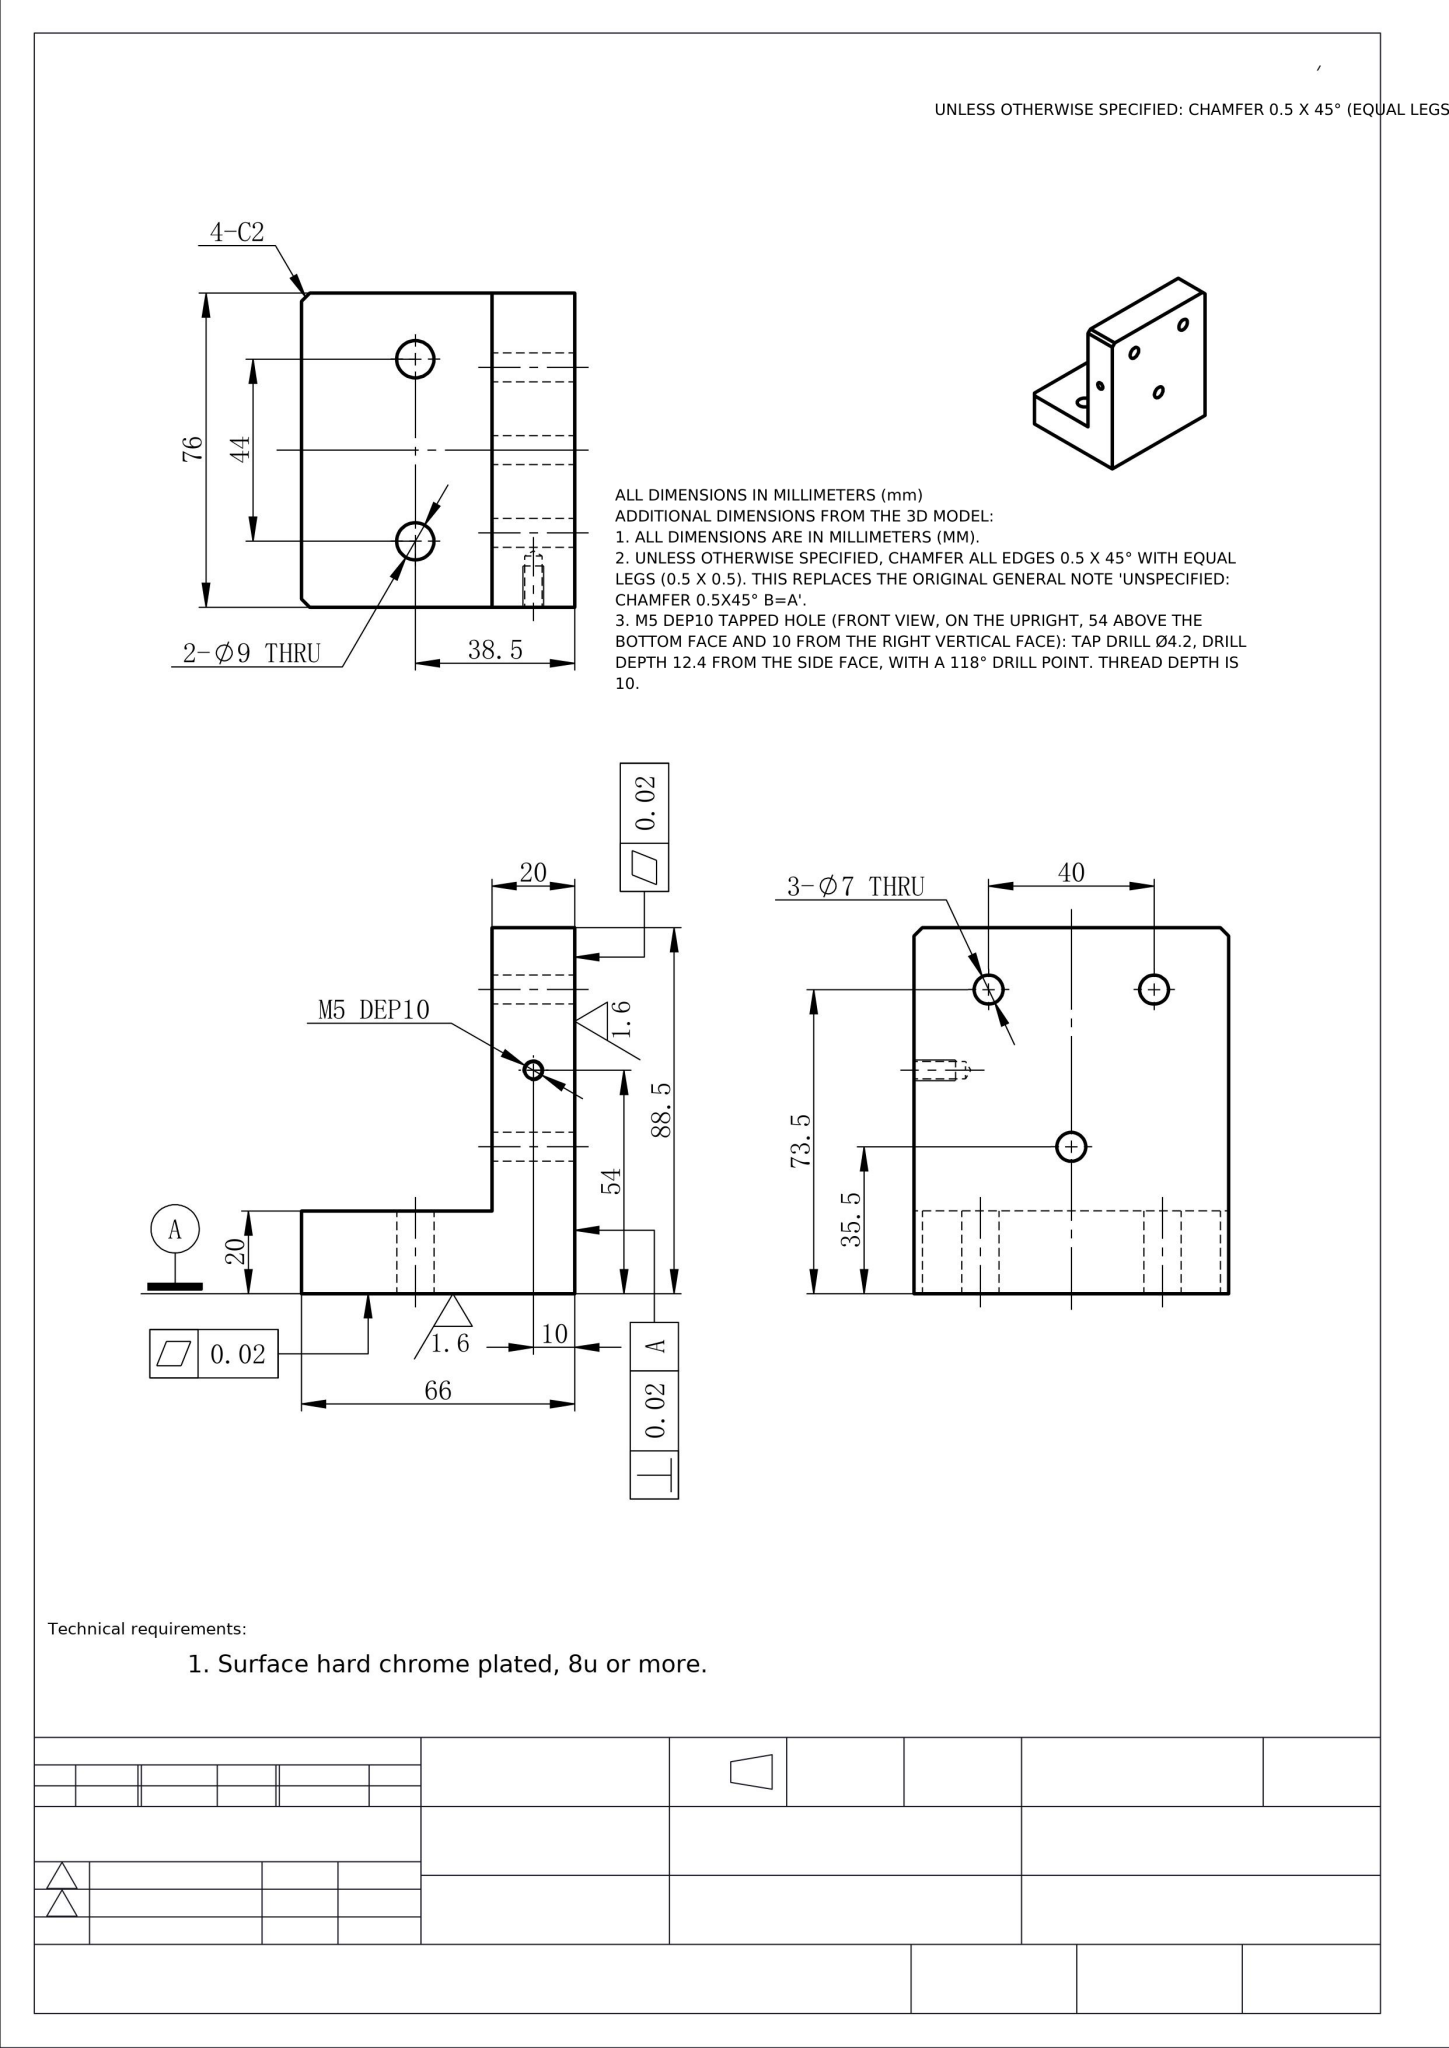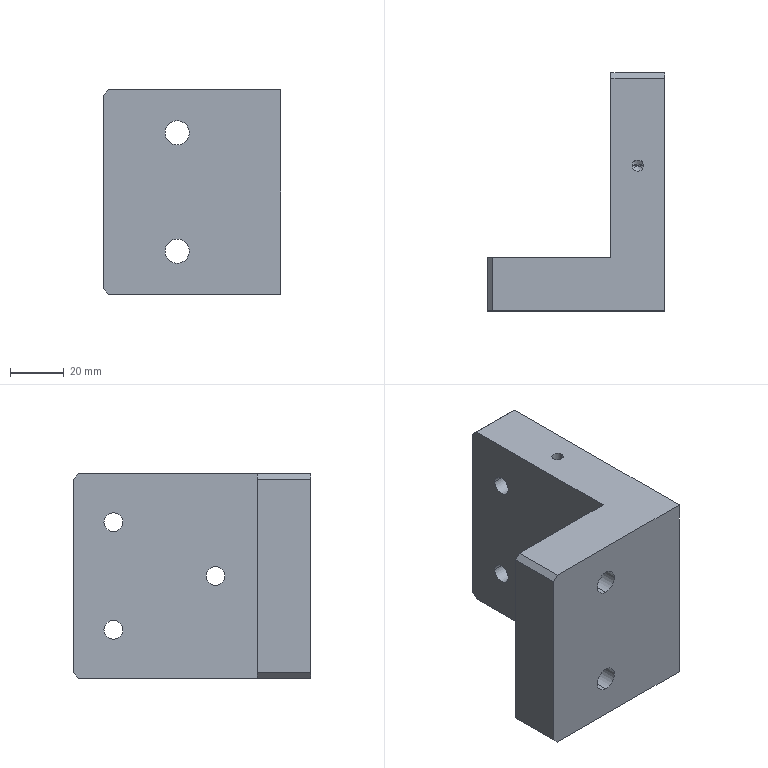Part | NX | mm | Five-Hole Corner Bracket | 1 solid | 26 faces | box 66 x 88.5 x 76 mm | volume 199249 mm3 | cylinder 12 | plane 12 | cone 2 | commonest cylinder face diameters 7 x6 9 x4 4.2 x2
STEP:
#1=COLOUR_RGB('',0.7961,0.8235,0.9373);
#2=FILL_AREA_STYLE_COLOUR('',#1);
#3=FILL_AREA_STYLE('',(#2));
#4=SURFACE_STYLE_FILL_AREA(#3);
#5=SURFACE_SIDE_STYLE('',(#4));
#6=SURFACE_STYLE_USAGE(.BOTH.,#5);
#7=PRESENTATION_STYLE_ASSIGNMENT((#6));
#8=CARTESIAN_POINT('',(-12.1,54.,25.6));
#9=VERTEX_POINT('',#8);
#10=CARTESIAN_POINT('',(-7.9,54.,25.6));
#11=VERTEX_POINT('',#10);
#12=CARTESIAN_POINT('',(-10.,54.,25.6));
#13=DIRECTION('',(0.,0.,1.));
#14=DIRECTION('',(1.,0.,0.));
#15=AXIS2_PLACEMENT_3D('',#12,#13,#14);
#16=CIRCLE('',#15,2.1);
#17=EDGE_CURVE('',#9,#11,#16,.T.);
#18=ORIENTED_EDGE('',*,*,#17,.F.);
#19=CARTESIAN_POINT('',(-12.1,54.,38.));
#20=VERTEX_POINT('',#19);
#21=CARTESIAN_POINT('',(-12.1,54.,38.));
#22=DIRECTION('',(0.,0.,1.));
#23=VECTOR('',#22,1000.);
#24=LINE('',#21,#23);
#25=EDGE_CURVE('',#9,#20,#24,.T.);
#26=ORIENTED_EDGE('',*,*,#25,.T.);
#27=CARTESIAN_POINT('',(-7.9,54.,38.));
#28=VERTEX_POINT('',#27);
#29=CARTESIAN_POINT('',(-10.,54.,38.));
#30=DIRECTION('',(0.,0.,1.));
#31=DIRECTION('',(1.,0.,0.));
#32=AXIS2_PLACEMENT_3D('',#29,#30,#31);
#33=CIRCLE('',#32,2.1);
#34=EDGE_CURVE('',#20,#28,#33,.T.);
#35=ORIENTED_EDGE('',*,*,#34,.T.);
#36=CARTESIAN_POINT('',(-7.9,54.,38.));
#37=DIRECTION('',(0.,0.,1.));
#38=VECTOR('',#37,1000.);
#39=LINE('',#36,#38);
#40=EDGE_CURVE('',#11,#28,#39,.T.);
#41=ORIENTED_EDGE('',*,*,#40,.F.);
#42=EDGE_LOOP('',(#18,#26,#35,#41));
#43=FACE_OUTER_BOUND('',#42,.T.);
#44=CARTESIAN_POINT('',(-10.,54.,38.));
#45=DIRECTION('',(0.,0.,1.));
#46=DIRECTION('',(1.,0.,0.));
#47=AXIS2_PLACEMENT_3D('',#44,#45,#46);
#48=CYLINDRICAL_SURFACE('',#47,2.1);
#49=ADVANCED_FACE('',(#43),#48,.F.);
#50=STYLED_ITEM('',(#7),#49);
#51=(LENGTH_UNIT()NAMED_UNIT(*)SI_UNIT(.MILLI.,.METRE.));
#52=UNCERTAINTY_MEASURE_WITH_UNIT(LENGTH_MEASURE(0.00001),#51,'','');
#53=(NAMED_UNIT(*)PLANE_ANGLE_UNIT()SI_UNIT($,.RADIAN.));
#54=(NAMED_UNIT(*)SI_UNIT($,.STERADIAN.)SOLID_ANGLE_UNIT());
#55=(GEOMETRIC_REPRESENTATION_CONTEXT(3)GLOBAL_UNCERTAINTY_ASSIGNED_CONTEXT((#52))GLOBAL_UNIT_ASSIGNED_CONTEXT((#51,#53,#54))REPRESENTATION_CONTEXT('',''));
#56=MECHANICAL_DESIGN_GEOMETRIC_PRESENTATION_REPRESENTATION('',(#50),#55);
#57=COLOUR_RGB('',0.7961,0.8235,0.9373);
#58=FILL_AREA_STYLE_COLOUR('',#57);
#59=FILL_AREA_STYLE('',(#58));
#60=SURFACE_STYLE_FILL_AREA(#59);
#61=SURFACE_SIDE_STYLE('',(#60));
#62=SURFACE_STYLE_USAGE(.BOTH.,#61);
#63=PRESENTATION_STYLE_ASSIGNMENT((#62));
#64=ORIENTED_EDGE('',*,*,#25,.F.);
#65=CARTESIAN_POINT('',(-10.,54.,25.6));
#66=DIRECTION('',(0.,0.,1.));
#67=DIRECTION('',(1.,0.,0.));
#68=AXIS2_PLACEMENT_3D('',#65,#66,#67);
#69=CIRCLE('',#68,2.1);
#70=EDGE_CURVE('',#11,#9,#69,.T.);
#71=ORIENTED_EDGE('',*,*,#70,.F.);
#72=ORIENTED_EDGE('',*,*,#40,.T.);
#73=CARTESIAN_POINT('',(-10.,54.,38.));
#74=DIRECTION('',(0.,0.,1.));
#75=DIRECTION('',(1.,0.,0.));
#76=AXIS2_PLACEMENT_3D('',#73,#74,#75);
#77=CIRCLE('',#76,2.1);
#78=EDGE_CURVE('',#28,#20,#77,.T.);
#79=ORIENTED_EDGE('',*,*,#78,.T.);
#80=EDGE_LOOP('',(#64,#71,#72,#79));
#81=FACE_OUTER_BOUND('',#80,.T.);
#82=CARTESIAN_POINT('',(-10.,54.,38.));
#83=DIRECTION('',(0.,0.,1.));
#84=DIRECTION('',(1.,0.,0.));
#85=AXIS2_PLACEMENT_3D('',#82,#83,#84);
#86=CYLINDRICAL_SURFACE('',#85,2.1);
#87=ADVANCED_FACE('',(#81),#86,.F.);
#88=STYLED_ITEM('',(#63),#87);
#89=(LENGTH_UNIT()NAMED_UNIT(*)SI_UNIT(.MILLI.,.METRE.));
#90=UNCERTAINTY_MEASURE_WITH_UNIT(LENGTH_MEASURE(0.00001),#89,'','');
#91=(NAMED_UNIT(*)PLANE_ANGLE_UNIT()SI_UNIT($,.RADIAN.));
#92=(NAMED_UNIT(*)SI_UNIT($,.STERADIAN.)SOLID_ANGLE_UNIT());
#93=(GEOMETRIC_REPRESENTATION_CONTEXT(3)GLOBAL_UNCERTAINTY_ASSIGNED_CONTEXT((#90))GLOBAL_UNIT_ASSIGNED_CONTEXT((#89,#91,#92))REPRESENTATION_CONTEXT('',''));
#94=MECHANICAL_DESIGN_GEOMETRIC_PRESENTATION_REPRESENTATION('',(#88),#93);
#95=PRESENTATION_LAYER_ASSIGNMENT('','',(#50));
#96=COLOUR_RGB('',0.7961,0.8235,0.9373);
#97=FILL_AREA_STYLE_COLOUR('',#96);
#98=FILL_AREA_STYLE('',(#97));
#99=SURFACE_STYLE_FILL_AREA(#98);
#100=SURFACE_SIDE_STYLE('',(#99));
#101=SURFACE_STYLE_USAGE(.BOTH.,#100);
#102=PRESENTATION_STYLE_ASSIGNMENT((#101));
#103=CARTESIAN_POINT('',(-10.,54.,24.338));
#104=VERTEX_POINT('',#103);
#105=CARTESIAN_POINT('',(-7.9,54.,25.6));
#106=DIRECTION('',(0.8572,0.,0.515));
#107=VECTOR('',#106,1000.);
#108=LINE('',#105,#107);
#109=EDGE_CURVE('',#104,#11,#108,.T.);
#110=ORIENTED_EDGE('',*,*,#109,.F.);
#111=CARTESIAN_POINT('',(-12.1,54.,25.6));
#112=DIRECTION('',(-0.8572,0.,0.515));
#113=VECTOR('',#112,1000.);
#114=LINE('',#111,#113);
#115=EDGE_CURVE('',#104,#9,#114,.T.);
#116=ORIENTED_EDGE('',*,*,#115,.T.);
#117=ORIENTED_EDGE('',*,*,#17,.T.);
#118=EDGE_LOOP('',(#110,#116,#117));
#119=FACE_OUTER_BOUND('',#118,.T.);
#120=CARTESIAN_POINT('',(-10.,54.,25.6));
#121=DIRECTION('',(0.,0.,1.));
#122=DIRECTION('',(1.,0.,0.));
#123=AXIS2_PLACEMENT_3D('',#120,#121,#122);
#124=CONICAL_SURFACE('',#123,2.1,1.03);
#125=ADVANCED_FACE('',(#119),#124,.F.);
#126=CARTESIAN_POINT('',(-20.,70.,-20.));
#127=VERTEX_POINT('',#126);
#128=CARTESIAN_POINT('',(-20.,77.,-20.));
#129=VERTEX_POINT('',#128);
#130=CARTESIAN_POINT('',(-20.,73.5,-20.));
#131=DIRECTION('',(1.,0.,0.));
#132=DIRECTION('',(0.,1.,0.));
#133=AXIS2_PLACEMENT_3D('',#130,#131,#132);
#134=CIRCLE('',#133,3.5);
#135=EDGE_CURVE('',#127,#129,#134,.T.);
#136=ORIENTED_EDGE('',*,*,#135,.F.);
#137=CARTESIAN_POINT('',(-0.,70.,-20.));
#138=VERTEX_POINT('',#137);
#139=CARTESIAN_POINT('',(-66.,70.,-20.));
#140=DIRECTION('',(1.,0.,0.));
#141=VECTOR('',#140,1000.);
#142=LINE('',#139,#141);
#143=EDGE_CURVE('',#127,#138,#142,.T.);
#144=ORIENTED_EDGE('',*,*,#143,.T.);
#145=CARTESIAN_POINT('',(-0.,77.,-20.));
#146=VERTEX_POINT('',#145);
#147=CARTESIAN_POINT('',(-0.,73.5,-20.));
#148=DIRECTION('',(1.,0.,0.));
#149=DIRECTION('',(-0.,1.,0.));
#150=AXIS2_PLACEMENT_3D('',#147,#148,#149);
#151=CIRCLE('',#150,3.5);
#152=EDGE_CURVE('',#138,#146,#151,.T.);
#153=ORIENTED_EDGE('',*,*,#152,.T.);
#154=CARTESIAN_POINT('',(-66.,77.,-20.));
#155=DIRECTION('',(1.,0.,0.));
#156=VECTOR('',#155,1000.);
#157=LINE('',#154,#156);
#158=EDGE_CURVE('',#129,#146,#157,.T.);
#159=ORIENTED_EDGE('',*,*,#158,.F.);
#160=EDGE_LOOP('',(#136,#144,#153,#159));
#161=FACE_OUTER_BOUND('',#160,.T.);
#162=CARTESIAN_POINT('',(-66.,73.5,-20.));
#163=DIRECTION('',(1.,0.,0.));
#164=DIRECTION('',(0.,1.,0.));
#165=AXIS2_PLACEMENT_3D('',#162,#163,#164);
#166=CYLINDRICAL_SURFACE('',#165,3.5);
#167=ADVANCED_FACE('',(#161),#166,.F.);
#168=CARTESIAN_POINT('',(-20.,70.,20.));
#169=VERTEX_POINT('',#168);
#170=CARTESIAN_POINT('',(-20.,77.,20.));
#171=VERTEX_POINT('',#170);
#172=CARTESIAN_POINT('',(-20.,73.5,20.));
#173=DIRECTION('',(1.,0.,0.));
#174=DIRECTION('',(0.,1.,0.));
#175=AXIS2_PLACEMENT_3D('',#172,#173,#174);
#176=CIRCLE('',#175,3.5);
#177=EDGE_CURVE('',#169,#171,#176,.T.);
#178=ORIENTED_EDGE('',*,*,#177,.F.);
#179=CARTESIAN_POINT('',(-0.,70.,20.));
#180=VERTEX_POINT('',#179);
#181=CARTESIAN_POINT('',(-66.,70.,20.));
#182=DIRECTION('',(1.,0.,0.));
#183=VECTOR('',#182,1000.);
#184=LINE('',#181,#183);
#185=EDGE_CURVE('',#169,#180,#184,.T.);
#186=ORIENTED_EDGE('',*,*,#185,.T.);
#187=CARTESIAN_POINT('',(-0.,77.,20.));
#188=VERTEX_POINT('',#187);
#189=CARTESIAN_POINT('',(-0.,73.5,20.));
#190=DIRECTION('',(1.,0.,0.));
#191=DIRECTION('',(-0.,1.,0.));
#192=AXIS2_PLACEMENT_3D('',#189,#190,#191);
#193=CIRCLE('',#192,3.5);
#194=EDGE_CURVE('',#180,#188,#193,.T.);
#195=ORIENTED_EDGE('',*,*,#194,.T.);
#196=CARTESIAN_POINT('',(-66.,77.,20.));
#197=DIRECTION('',(1.,0.,0.));
#198=VECTOR('',#197,1000.);
#199=LINE('',#196,#198);
#200=EDGE_CURVE('',#171,#188,#199,.T.);
#201=ORIENTED_EDGE('',*,*,#200,.F.);
#202=EDGE_LOOP('',(#178,#186,#195,#201));
#203=FACE_OUTER_BOUND('',#202,.T.);
#204=CARTESIAN_POINT('',(-66.,73.5,20.));
#205=DIRECTION('',(1.,0.,0.));
#206=DIRECTION('',(0.,1.,0.));
#207=AXIS2_PLACEMENT_3D('',#204,#205,#206);
#208=CYLINDRICAL_SURFACE('',#207,3.5);
#209=ADVANCED_FACE('',(#203),#208,.F.);
#210=CARTESIAN_POINT('',(-20.,32.,0.));
#211=VERTEX_POINT('',#210);
#212=CARTESIAN_POINT('',(-20.,39.,0.));
#213=VERTEX_POINT('',#212);
#214=CARTESIAN_POINT('',(-20.,35.5,0.));
#215=DIRECTION('',(1.,0.,0.));
#216=DIRECTION('',(0.,1.,0.));
#217=AXIS2_PLACEMENT_3D('',#214,#215,#216);
#218=CIRCLE('',#217,3.5);
#219=EDGE_CURVE('',#211,#213,#218,.T.);
#220=ORIENTED_EDGE('',*,*,#219,.F.);
#221=CARTESIAN_POINT('',(-0.,32.,0.));
#222=VERTEX_POINT('',#221);
#223=CARTESIAN_POINT('',(-66.,32.,0.));
#224=DIRECTION('',(1.,0.,0.));
#225=VECTOR('',#224,1000.);
#226=LINE('',#223,#225);
#227=EDGE_CURVE('',#211,#222,#226,.T.);
#228=ORIENTED_EDGE('',*,*,#227,.T.);
#229=CARTESIAN_POINT('',(-0.,39.,0.));
#230=VERTEX_POINT('',#229);
#231=CARTESIAN_POINT('',(-0.,35.5,0.));
#232=DIRECTION('',(1.,0.,0.));
#233=DIRECTION('',(-0.,1.,0.));
#234=AXIS2_PLACEMENT_3D('',#231,#232,#233);
#235=CIRCLE('',#234,3.5);
#236=EDGE_CURVE('',#222,#230,#235,.T.);
#237=ORIENTED_EDGE('',*,*,#236,.T.);
#238=CARTESIAN_POINT('',(-66.,39.,0.));
#239=DIRECTION('',(1.,0.,0.));
#240=VECTOR('',#239,1000.);
#241=LINE('',#238,#240);
#242=EDGE_CURVE('',#213,#230,#241,.T.);
#243=ORIENTED_EDGE('',*,*,#242,.F.);
#244=EDGE_LOOP('',(#220,#228,#237,#243));
#245=FACE_OUTER_BOUND('',#244,.T.);
#246=CARTESIAN_POINT('',(-66.,35.5,0.));
#247=DIRECTION('',(1.,0.,0.));
#248=DIRECTION('',(0.,1.,0.));
#249=AXIS2_PLACEMENT_3D('',#246,#247,#248);
#250=CYLINDRICAL_SURFACE('',#249,3.5);
#251=ADVANCED_FACE('',(#245),#250,.F.);
#252=CARTESIAN_POINT('',(-38.5,-0.,17.5));
#253=VERTEX_POINT('',#252);
#254=CARTESIAN_POINT('',(-38.5,-0.,26.5));
#255=VERTEX_POINT('',#254);
#256=CARTESIAN_POINT('',(-38.5,-0.,22.));
#257=DIRECTION('',(0.,1.,0.));
#258=DIRECTION('',(0.,0.,1.));
#259=AXIS2_PLACEMENT_3D('',#256,#257,#258);
#260=CIRCLE('',#259,4.5);
#261=EDGE_CURVE('',#253,#255,#260,.T.);
#262=ORIENTED_EDGE('',*,*,#261,.F.);
#263=CARTESIAN_POINT('',(-38.5,20.,17.5));
#264=VERTEX_POINT('',#263);
#265=CARTESIAN_POINT('',(-38.5,-0.,17.5));
#266=DIRECTION('',(0.,1.,0.));
#267=VECTOR('',#266,1000.);
#268=LINE('',#265,#267);
#269=EDGE_CURVE('',#253,#264,#268,.T.);
#270=ORIENTED_EDGE('',*,*,#269,.T.);
#271=CARTESIAN_POINT('',(-38.5,20.,26.5));
#272=VERTEX_POINT('',#271);
#273=CARTESIAN_POINT('',(-38.5,20.,22.));
#274=DIRECTION('',(0.,1.,0.));
#275=DIRECTION('',(0.,0.,1.));
#276=AXIS2_PLACEMENT_3D('',#273,#274,#275);
#277=CIRCLE('',#276,4.5);
#278=EDGE_CURVE('',#264,#272,#277,.T.);
#279=ORIENTED_EDGE('',*,*,#278,.T.);
#280=CARTESIAN_POINT('',(-38.5,-0.,26.5));
#281=DIRECTION('',(0.,1.,0.));
#282=VECTOR('',#281,1000.);
#283=LINE('',#280,#282);
#284=EDGE_CURVE('',#255,#272,#283,.T.);
#285=ORIENTED_EDGE('',*,*,#284,.F.);
#286=EDGE_LOOP('',(#262,#270,#279,#285));
#287=FACE_OUTER_BOUND('',#286,.T.);
#288=CARTESIAN_POINT('',(-38.5,-0.,22.));
#289=DIRECTION('',(0.,1.,0.));
#290=DIRECTION('',(0.,0.,1.));
#291=AXIS2_PLACEMENT_3D('',#288,#289,#290);
#292=CYLINDRICAL_SURFACE('',#291,4.5);
#293=ADVANCED_FACE('',(#287),#292,.F.);
#294=CARTESIAN_POINT('',(-38.5,-0.,-26.5));
#295=VERTEX_POINT('',#294);
#296=CARTESIAN_POINT('',(-38.5,-0.,-17.5));
#297=VERTEX_POINT('',#296);
#298=CARTESIAN_POINT('',(-38.5,-0.,-22.));
#299=DIRECTION('',(0.,1.,0.));
#300=DIRECTION('',(0.,0.,1.));
#301=AXIS2_PLACEMENT_3D('',#298,#299,#300);
#302=CIRCLE('',#301,4.5);
#303=EDGE_CURVE('',#295,#297,#302,.T.);
#304=ORIENTED_EDGE('',*,*,#303,.F.);
#305=CARTESIAN_POINT('',(-38.5,20.,-26.5));
#306=VERTEX_POINT('',#305);
#307=CARTESIAN_POINT('',(-38.5,-0.,-26.5));
#308=DIRECTION('',(0.,1.,0.));
#309=VECTOR('',#308,1000.);
#310=LINE('',#307,#309);
#311=EDGE_CURVE('',#295,#306,#310,.T.);
#312=ORIENTED_EDGE('',*,*,#311,.T.);
#313=CARTESIAN_POINT('',(-38.5,20.,-17.5));
#314=VERTEX_POINT('',#313);
#315=CARTESIAN_POINT('',(-38.5,20.,-22.));
#316=DIRECTION('',(0.,1.,0.));
#317=DIRECTION('',(0.,0.,1.));
#318=AXIS2_PLACEMENT_3D('',#315,#316,#317);
#319=CIRCLE('',#318,4.5);
#320=EDGE_CURVE('',#306,#314,#319,.T.);
#321=ORIENTED_EDGE('',*,*,#320,.T.);
#322=CARTESIAN_POINT('',(-38.5,-0.,-17.5));
#323=DIRECTION('',(0.,1.,0.));
#324=VECTOR('',#323,1000.);
#325=LINE('',#322,#324);
#326=EDGE_CURVE('',#297,#314,#325,.T.);
#327=ORIENTED_EDGE('',*,*,#326,.F.);
#328=EDGE_LOOP('',(#304,#312,#321,#327));
#329=FACE_OUTER_BOUND('',#328,.T.);
#330=CARTESIAN_POINT('',(-38.5,-0.,-22.));
#331=DIRECTION('',(0.,1.,0.));
#332=DIRECTION('',(0.,0.,1.));
#333=AXIS2_PLACEMENT_3D('',#330,#331,#332);
#334=CYLINDRICAL_SURFACE('',#333,4.5);
#335=ADVANCED_FACE('',(#329),#334,.F.);
#336=CARTESIAN_POINT('',(-0.,73.5,-20.));
#337=DIRECTION('',(1.,0.,0.));
#338=DIRECTION('',(-0.,1.,0.));
#339=AXIS2_PLACEMENT_3D('',#336,#337,#338);
#340=CIRCLE('',#339,3.5);
#341=EDGE_CURVE('',#146,#138,#340,.T.);
#342=ORIENTED_EDGE('',*,*,#341,.F.);
#343=ORIENTED_EDGE('',*,*,#152,.F.);
#344=EDGE_LOOP('',(#342,#343));
#345=FACE_BOUND('',#344,.T.);
#346=CARTESIAN_POINT('',(-0.,73.5,20.));
#347=DIRECTION('',(1.,0.,0.));
#348=DIRECTION('',(-0.,1.,0.));
#349=AXIS2_PLACEMENT_3D('',#346,#347,#348);
#350=CIRCLE('',#349,3.5);
#351=EDGE_CURVE('',#188,#180,#350,.T.);
#352=ORIENTED_EDGE('',*,*,#351,.F.);
#353=ORIENTED_EDGE('',*,*,#194,.F.);
#354=EDGE_LOOP('',(#352,#353));
#355=FACE_BOUND('',#354,.T.);
#356=CARTESIAN_POINT('',(-0.,35.5,0.));
#357=DIRECTION('',(1.,0.,0.));
#358=DIRECTION('',(-0.,1.,0.));
#359=AXIS2_PLACEMENT_3D('',#356,#357,#358);
#360=CIRCLE('',#359,3.5);
#361=EDGE_CURVE('',#230,#222,#360,.T.);
#362=ORIENTED_EDGE('',*,*,#361,.F.);
#363=ORIENTED_EDGE('',*,*,#236,.F.);
#364=EDGE_LOOP('',(#362,#363));
#365=FACE_BOUND('',#364,.T.);
#366=CARTESIAN_POINT('',(0.,0.,-38.));
#367=VERTEX_POINT('',#366);
#368=CARTESIAN_POINT('',(-0.,86.5,-38.));
#369=VERTEX_POINT('',#368);
#370=CARTESIAN_POINT('',(0.,0.,-38.));
#371=DIRECTION('',(-0.,1.,0.));
#372=VECTOR('',#371,1000.);
#373=LINE('',#370,#372);
#374=EDGE_CURVE('',#367,#369,#373,.T.);
#375=ORIENTED_EDGE('',*,*,#374,.T.);
#376=CARTESIAN_POINT('',(-0.,88.5,-36.));
#377=VERTEX_POINT('',#376);
#378=CARTESIAN_POINT('',(-0.,88.5,-36.));
#379=DIRECTION('',(-0.,0.7071,0.7071));
#380=VECTOR('',#379,1000.);
#381=LINE('',#378,#380);
#382=EDGE_CURVE('',#369,#377,#381,.T.);
#383=ORIENTED_EDGE('',*,*,#382,.T.);
#384=CARTESIAN_POINT('',(-0.,88.5,36.));
#385=VERTEX_POINT('',#384);
#386=CARTESIAN_POINT('',(-0.,88.5,38.));
#387=DIRECTION('',(0.,0.,-1.));
#388=VECTOR('',#387,1000.);
#389=LINE('',#386,#388);
#390=EDGE_CURVE('',#385,#377,#389,.T.);
#391=ORIENTED_EDGE('',*,*,#390,.F.);
#392=CARTESIAN_POINT('',(-0.,86.5,38.));
#393=VERTEX_POINT('',#392);
#394=CARTESIAN_POINT('',(-0.,86.5,38.));
#395=DIRECTION('',(0.,-0.7071,0.7071));
#396=VECTOR('',#395,1000.);
#397=LINE('',#394,#396);
#398=EDGE_CURVE('',#385,#393,#397,.T.);
#399=ORIENTED_EDGE('',*,*,#398,.T.);
#400=CARTESIAN_POINT('',(0.,0.,38.));
#401=VERTEX_POINT('',#400);
#402=CARTESIAN_POINT('',(0.,0.,38.));
#403=DIRECTION('',(-0.,1.,0.));
#404=VECTOR('',#403,1000.);
#405=LINE('',#402,#404);
#406=EDGE_CURVE('',#401,#393,#405,.T.);
#407=ORIENTED_EDGE('',*,*,#406,.F.);
#408=CARTESIAN_POINT('',(0.,0.,38.));
#409=DIRECTION('',(0.,0.,-1.));
#410=VECTOR('',#409,1000.);
#411=LINE('',#408,#410);
#412=EDGE_CURVE('',#401,#367,#411,.T.);
#413=ORIENTED_EDGE('',*,*,#412,.T.);
#414=EDGE_LOOP('',(#375,#383,#391,#399,#407,#413));
#415=FACE_OUTER_BOUND('',#414,.T.);
#416=CARTESIAN_POINT('',(0.,0.,38.));
#417=DIRECTION('',(-1.,-0.,0.));
#418=DIRECTION('',(0.,-1.,0.));
#419=AXIS2_PLACEMENT_3D('',#416,#417,#418);
#420=PLANE('',#419);
#421=ADVANCED_FACE('',(#345,#355,#365,#415),#420,.F.);
#422=ORIENTED_EDGE('',*,*,#390,.T.);
#423=CARTESIAN_POINT('',(-20.,88.5,-36.));
#424=VERTEX_POINT('',#423);
#425=CARTESIAN_POINT('',(-20.,88.5,-36.));
#426=DIRECTION('',(-1.,0.,0.));
#427=VECTOR('',#426,1000.);
#428=LINE('',#425,#427);
#429=EDGE_CURVE('',#377,#424,#428,.T.);
#430=ORIENTED_EDGE('',*,*,#429,.T.);
#431=CARTESIAN_POINT('',(-20.,88.5,36.));
#432=VERTEX_POINT('',#431);
#433=CARTESIAN_POINT('',(-20.,88.5,38.));
#434=DIRECTION('',(0.,0.,-1.));
#435=VECTOR('',#434,1000.);
#436=LINE('',#433,#435);
#437=EDGE_CURVE('',#432,#424,#436,.T.);
#438=ORIENTED_EDGE('',*,*,#437,.F.);
#439=CARTESIAN_POINT('',(-20.,88.5,36.));
#440=DIRECTION('',(1.,0.,0.));
#441=VECTOR('',#440,1000.);
#442=LINE('',#439,#441);
#443=EDGE_CURVE('',#432,#385,#442,.T.);
#444=ORIENTED_EDGE('',*,*,#443,.T.);
#445=EDGE_LOOP('',(#422,#430,#438,#444));
#446=FACE_OUTER_BOUND('',#445,.T.);
#447=CARTESIAN_POINT('',(-20.,88.5,38.));
#448=DIRECTION('',(0.,-1.,0.));
#449=DIRECTION('',(0.,0.,-1.));
#450=AXIS2_PLACEMENT_3D('',#447,#448,#449);
#451=PLANE('',#450);
#452=ADVANCED_FACE('',(#446),#451,.F.);
#453=CARTESIAN_POINT('',(-20.,73.5,-20.));
#454=DIRECTION('',(1.,0.,0.));
#455=DIRECTION('',(0.,1.,0.));
#456=AXIS2_PLACEMENT_3D('',#453,#454,#455);
#457=CIRCLE('',#456,3.5);
#458=EDGE_CURVE('',#129,#127,#457,.T.);
#459=ORIENTED_EDGE('',*,*,#458,.T.);
#460=ORIENTED_EDGE('',*,*,#135,.T.);
#461=EDGE_LOOP('',(#459,#460));
#462=FACE_BOUND('',#461,.T.);
#463=CARTESIAN_POINT('',(-20.,73.5,20.));
#464=DIRECTION('',(1.,0.,0.));
#465=DIRECTION('',(0.,1.,0.));
#466=AXIS2_PLACEMENT_3D('',#463,#464,#465);
#467=CIRCLE('',#466,3.5);
#468=EDGE_CURVE('',#171,#169,#467,.T.);
#469=ORIENTED_EDGE('',*,*,#468,.T.);
#470=ORIENTED_EDGE('',*,*,#177,.T.);
#471=EDGE_LOOP('',(#469,#470));
#472=FACE_BOUND('',#471,.T.);
#473=CARTESIAN_POINT('',(-20.,35.5,0.));
#474=DIRECTION('',(1.,0.,0.));
#475=DIRECTION('',(0.,1.,0.));
#476=AXIS2_PLACEMENT_3D('',#473,#474,#475);
#477=CIRCLE('',#476,3.5);
#478=EDGE_CURVE('',#213,#211,#477,.T.);
#479=ORIENTED_EDGE('',*,*,#478,.T.);
#480=ORIENTED_EDGE('',*,*,#219,.T.);
#481=EDGE_LOOP('',(#479,#480));
#482=FACE_BOUND('',#481,.T.);
#483=ORIENTED_EDGE('',*,*,#437,.T.);
#484=CARTESIAN_POINT('',(-20.,86.5,-38.));
#485=VERTEX_POINT('',#484);
#486=CARTESIAN_POINT('',(-20.,88.5,-36.));
#487=DIRECTION('',(0.,-0.7071,-0.7071));
#488=VECTOR('',#487,1000.);
#489=LINE('',#486,#488);
#490=EDGE_CURVE('',#424,#485,#489,.T.);
#491=ORIENTED_EDGE('',*,*,#490,.T.);
#492=CARTESIAN_POINT('',(-20.,20.,-38.));
#493=VERTEX_POINT('',#492);
#494=CARTESIAN_POINT('',(-20.,20.,-38.));
#495=DIRECTION('',(0.,-1.,0.));
#496=VECTOR('',#495,1000.);
#497=LINE('',#494,#496);
#498=EDGE_CURVE('',#485,#493,#497,.T.);
#499=ORIENTED_EDGE('',*,*,#498,.T.);
#500=CARTESIAN_POINT('',(-20.,20.,38.));
#501=VERTEX_POINT('',#500);
#502=CARTESIAN_POINT('',(-20.,20.,38.));
#503=DIRECTION('',(0.,0.,-1.));
#504=VECTOR('',#503,1000.);
#505=LINE('',#502,#504);
#506=EDGE_CURVE('',#501,#493,#505,.T.);
#507=ORIENTED_EDGE('',*,*,#506,.F.);
#508=CARTESIAN_POINT('',(-20.,86.5,38.));
#509=VERTEX_POINT('',#508);
#510=CARTESIAN_POINT('',(-20.,20.,38.));
#511=DIRECTION('',(0.,-1.,0.));
#512=VECTOR('',#511,1000.);
#513=LINE('',#510,#512);
#514=EDGE_CURVE('',#509,#501,#513,.T.);
#515=ORIENTED_EDGE('',*,*,#514,.F.);
#516=CARTESIAN_POINT('',(-20.,86.5,38.));
#517=DIRECTION('',(-0.,0.7071,-0.7071));
#518=VECTOR('',#517,1000.);
#519=LINE('',#516,#518);
#520=EDGE_CURVE('',#509,#432,#519,.T.);
#521=ORIENTED_EDGE('',*,*,#520,.T.);
#522=EDGE_LOOP('',(#483,#491,#499,#507,#515,#521));
#523=FACE_OUTER_BOUND('',#522,.T.);
#524=CARTESIAN_POINT('',(-20.,20.,38.));
#525=DIRECTION('',(1.,0.,0.));
#526=DIRECTION('',(-0.,1.,0.));
#527=AXIS2_PLACEMENT_3D('',#524,#525,#526);
#528=PLANE('',#527);
#529=ADVANCED_FACE('',(#462,#472,#482,#523),#528,.F.);
#530=CARTESIAN_POINT('',(-38.5,20.,22.));
#531=DIRECTION('',(0.,1.,0.));
#532=DIRECTION('',(0.,0.,1.));
#533=AXIS2_PLACEMENT_3D('',#530,#531,#532);
#534=CIRCLE('',#533,4.5);
#535=EDGE_CURVE('',#272,#264,#534,.T.);
#536=ORIENTED_EDGE('',*,*,#535,.F.);
#537=ORIENTED_EDGE('',*,*,#278,.F.);
#538=EDGE_LOOP('',(#536,#537));
#539=FACE_BOUND('',#538,.T.);
#540=CARTESIAN_POINT('',(-38.5,20.,-22.));
#541=DIRECTION('',(0.,1.,0.));
#542=DIRECTION('',(0.,0.,1.));
#543=AXIS2_PLACEMENT_3D('',#540,#541,#542);
#544=CIRCLE('',#543,4.5);
#545=EDGE_CURVE('',#314,#306,#544,.T.);
#546=ORIENTED_EDGE('',*,*,#545,.F.);
#547=ORIENTED_EDGE('',*,*,#320,.F.);
#548=EDGE_LOOP('',(#546,#547));
#549=FACE_BOUND('',#548,.T.);
#550=CARTESIAN_POINT('',(-66.,20.,36.));
#551=VERTEX_POINT('',#550);
#552=CARTESIAN_POINT('',(-66.,20.,-36.));
#553=VERTEX_POINT('',#552);
#554=CARTESIAN_POINT('',(-66.,20.,38.));
#555=DIRECTION('',(0.,0.,-1.));
#556=VECTOR('',#555,1000.);
#557=LINE('',#554,#556);
#558=EDGE_CURVE('',#551,#553,#557,.T.);
#559=ORIENTED_EDGE('',*,*,#558,.F.);
#560=CARTESIAN_POINT('',(-64.,20.,38.));
#561=VERTEX_POINT('',#560);
#562=CARTESIAN_POINT('',(-64.,20.,38.));
#563=DIRECTION('',(0.7071,0.,0.7071));
#564=VECTOR('',#563,1000.);
#565=LINE('',#562,#564);
#566=EDGE_CURVE('',#551,#561,#565,.T.);
#567=ORIENTED_EDGE('',*,*,#566,.T.);
#568=CARTESIAN_POINT('',(-66.,20.,38.));
#569=DIRECTION('',(-1.,0.,0.));
#570=VECTOR('',#569,1000.);
#571=LINE('',#568,#570);
#572=EDGE_CURVE('',#501,#561,#571,.T.);
#573=ORIENTED_EDGE('',*,*,#572,.F.);
#574=ORIENTED_EDGE('',*,*,#506,.T.);
#575=CARTESIAN_POINT('',(-64.,20.,-38.));
#576=VERTEX_POINT('',#575);
#577=CARTESIAN_POINT('',(-66.,20.,-38.));
#578=DIRECTION('',(-1.,0.,0.));
#579=VECTOR('',#578,1000.);
#580=LINE('',#577,#579);
#581=EDGE_CURVE('',#493,#576,#580,.T.);
#582=ORIENTED_EDGE('',*,*,#581,.T.);
#583=CARTESIAN_POINT('',(-66.,20.,-36.));
#584=DIRECTION('',(-0.7071,0.,0.7071));
#585=VECTOR('',#584,1000.);
#586=LINE('',#583,#585);
#587=EDGE_CURVE('',#576,#553,#586,.T.);
#588=ORIENTED_EDGE('',*,*,#587,.T.);
#589=EDGE_LOOP('',(#559,#567,#573,#574,#582,#588));
#590=FACE_OUTER_BOUND('',#589,.T.);
#591=CARTESIAN_POINT('',(-66.,20.,38.));
#592=DIRECTION('',(0.,-1.,0.));
#593=DIRECTION('',(0.,0.,-1.));
#594=AXIS2_PLACEMENT_3D('',#591,#592,#593);
#595=PLANE('',#594);
#596=ADVANCED_FACE('',(#539,#549,#590),#595,.F.);
#597=CARTESIAN_POINT('',(-66.,-0.,36.));
#598=VERTEX_POINT('',#597);
#599=CARTESIAN_POINT('',(-66.,-0.,-36.));
#600=VERTEX_POINT('',#599);
#601=CARTESIAN_POINT('',(-66.,-0.,38.));
#602=DIRECTION('',(0.,0.,-1.));
#603=VECTOR('',#602,1000.);
#604=LINE('',#601,#603);
#605=EDGE_CURVE('',#598,#600,#604,.T.);
#606=ORIENTED_EDGE('',*,*,#605,.F.);
#607=CARTESIAN_POINT('',(-66.,-0.,36.));
#608=DIRECTION('',(0.,1.,0.));
#609=VECTOR('',#608,1000.);
#610=LINE('',#607,#609);
#611=EDGE_CURVE('',#598,#551,#610,.T.);
#612=ORIENTED_EDGE('',*,*,#611,.T.);
#613=ORIENTED_EDGE('',*,*,#558,.T.);
#614=CARTESIAN_POINT('',(-66.,-0.,-36.));
#615=DIRECTION('',(0.,-1.,0.));
#616=VECTOR('',#615,1000.);
#617=LINE('',#614,#616);
#618=EDGE_CURVE('',#553,#600,#617,.T.);
#619=ORIENTED_EDGE('',*,*,#618,.T.);
#620=EDGE_LOOP('',(#606,#612,#613,#619));
#621=FACE_OUTER_BOUND('',#620,.T.);
#622=CARTESIAN_POINT('',(-66.,-0.,38.));
#623=DIRECTION('',(1.,0.,0.));
#624=DIRECTION('',(0.,0.,-1.));
#625=AXIS2_PLACEMENT_3D('',#622,#623,#624);
#626=PLANE('',#625);
#627=ADVANCED_FACE('',(#621),#626,.F.);
#628=CARTESIAN_POINT('',(-38.5,-0.,22.));
#629=DIRECTION('',(0.,1.,0.));
#630=DIRECTION('',(0.,0.,1.));
#631=AXIS2_PLACEMENT_3D('',#628,#629,#630);
#632=CIRCLE('',#631,4.5);
#633=EDGE_CURVE('',#255,#253,#632,.T.);
#634=ORIENTED_EDGE('',*,*,#633,.T.);
#635=ORIENTED_EDGE('',*,*,#261,.T.);
#636=EDGE_LOOP('',(#634,#635));
#637=FACE_BOUND('',#636,.T.);
#638=CARTESIAN_POINT('',(-38.5,-0.,-22.));
#639=DIRECTION('',(0.,1.,0.));
#640=DIRECTION('',(0.,0.,1.));
#641=AXIS2_PLACEMENT_3D('',#638,#639,#640);
#642=CIRCLE('',#641,4.5);
#643=EDGE_CURVE('',#297,#295,#642,.T.);
#644=ORIENTED_EDGE('',*,*,#643,.T.);
#645=ORIENTED_EDGE('',*,*,#303,.T.);
#646=EDGE_LOOP('',(#644,#645));
#647=FACE_BOUND('',#646,.T.);
#648=CARTESIAN_POINT('',(-64.,-0.,38.));
#649=VERTEX_POINT('',#648);
#650=CARTESIAN_POINT('',(0.,0.,38.));
#651=DIRECTION('',(1.,0.,0.));
#652=VECTOR('',#651,1000.);
#653=LINE('',#650,#652);
#654=EDGE_CURVE('',#649,#401,#653,.T.);
#655=ORIENTED_EDGE('',*,*,#654,.F.);
#656=CARTESIAN_POINT('',(-64.,-0.,38.));
#657=DIRECTION('',(-0.7071,-0.,-0.7071));
#658=VECTOR('',#657,1000.);
#659=LINE('',#656,#658);
#660=EDGE_CURVE('',#649,#598,#659,.T.);
#661=ORIENTED_EDGE('',*,*,#660,.T.);
#662=ORIENTED_EDGE('',*,*,#605,.T.);
#663=CARTESIAN_POINT('',(-64.,-0.,-38.));
#664=VERTEX_POINT('',#663);
#665=CARTESIAN_POINT('',(-66.,-0.,-36.));
#666=DIRECTION('',(0.7071,0.,-0.7071));
#667=VECTOR('',#666,1000.);
#668=LINE('',#665,#667);
#669=EDGE_CURVE('',#600,#664,#668,.T.);
#670=ORIENTED_EDGE('',*,*,#669,.T.);
#671=CARTESIAN_POINT('',(0.,0.,-38.));
#672=DIRECTION('',(1.,0.,0.));
#673=VECTOR('',#672,1000.);
#674=LINE('',#671,#673);
#675=EDGE_CURVE('',#664,#367,#674,.T.);
#676=ORIENTED_EDGE('',*,*,#675,.T.);
#677=ORIENTED_EDGE('',*,*,#412,.F.);
#678=EDGE_LOOP('',(#655,#661,#662,#670,#676,#677));
#679=FACE_OUTER_BOUND('',#678,.T.);
#680=CARTESIAN_POINT('',(0.,0.,38.));
#681=DIRECTION('',(-0.,1.,0.));
#682=DIRECTION('',(-1.,-0.,0.));
#683=AXIS2_PLACEMENT_3D('',#680,#681,#682);
#684=PLANE('',#683);
#685=ADVANCED_FACE('',(#637,#647,#679),#684,.F.);
#686=ORIENTED_EDGE('',*,*,#78,.F.);
#687=ORIENTED_EDGE('',*,*,#34,.F.);
#688=EDGE_LOOP('',(#686,#687));
#689=FACE_BOUND('',#688,.T.);
#690=ORIENTED_EDGE('',*,*,#406,.T.);
#691=CARTESIAN_POINT('',(-0.,86.5,38.));
#692=DIRECTION('',(-1.,0.,0.));
#693=VECTOR('',#692,1000.);
#694=LINE('',#691,#693);
#695=EDGE_CURVE('',#393,#509,#694,.T.);
#696=ORIENTED_EDGE('',*,*,#695,.T.);
#697=ORIENTED_EDGE('',*,*,#514,.T.);
#698=ORIENTED_EDGE('',*,*,#572,.T.);
#699=CARTESIAN_POINT('',(-64.,88.5,38.));
#700=DIRECTION('',(0.,-1.,0.));
#701=VECTOR('',#700,1000.);
#702=LINE('',#699,#701);
#703=EDGE_CURVE('',#561,#649,#702,.T.);
#704=ORIENTED_EDGE('',*,*,#703,.T.);
#705=ORIENTED_EDGE('',*,*,#654,.T.);
#706=EDGE_LOOP('',(#690,#696,#697,#698,#704,#705));
#707=FACE_OUTER_BOUND('',#706,.T.);
#708=CARTESIAN_POINT('',(-0.,88.5,38.));
#709=DIRECTION('',(0.,0.,-1.));
#710=DIRECTION('',(-1.,0.,0.));
#711=AXIS2_PLACEMENT_3D('',#708,#709,#710);
#712=PLANE('',#711);
#713=ADVANCED_FACE('',(#689,#707),#712,.F.);
#714=ORIENTED_EDGE('',*,*,#498,.F.);
#715=CARTESIAN_POINT('',(-0.,86.5,-38.));
#716=DIRECTION('',(1.,0.,0.));
#717=VECTOR('',#716,1000.);
#718=LINE('',#715,#717);
#719=EDGE_CURVE('',#485,#369,#718,.T.);
#720=ORIENTED_EDGE('',*,*,#719,.T.);
#721=ORIENTED_EDGE('',*,*,#374,.F.);
#722=ORIENTED_EDGE('',*,*,#675,.F.);
#723=CARTESIAN_POINT('',(-64.,20.,-38.));
#724=DIRECTION('',(0.,1.,0.));
#725=VECTOR('',#724,1000.);
#726=LINE('',#723,#725);
#727=EDGE_CURVE('',#664,#576,#726,.T.);
#728=ORIENTED_EDGE('',*,*,#727,.T.);
#729=ORIENTED_EDGE('',*,*,#581,.F.);
#730=EDGE_LOOP('',(#714,#720,#721,#722,#728,#729));
#731=FACE_OUTER_BOUND('',#730,.T.);
#732=CARTESIAN_POINT('',(-0.,88.5,-38.));
#733=DIRECTION('',(0.,0.,-1.));
#734=DIRECTION('',(-1.,0.,0.));
#735=AXIS2_PLACEMENT_3D('',#732,#733,#734);
#736=PLANE('',#735);
#737=ADVANCED_FACE('',(#731),#736,.T.);
#738=ORIENTED_EDGE('',*,*,#311,.F.);
#739=ORIENTED_EDGE('',*,*,#643,.F.);
#740=ORIENTED_EDGE('',*,*,#326,.T.);
#741=ORIENTED_EDGE('',*,*,#545,.T.);
#742=EDGE_LOOP('',(#738,#739,#740,#741));
#743=FACE_OUTER_BOUND('',#742,.T.);
#744=CARTESIAN_POINT('',(-38.5,-0.,-22.));
#745=DIRECTION('',(0.,1.,0.));
#746=DIRECTION('',(0.,0.,1.));
#747=AXIS2_PLACEMENT_3D('',#744,#745,#746);
#748=CYLINDRICAL_SURFACE('',#747,4.5);
#749=ADVANCED_FACE('',(#743),#748,.F.);
#750=ORIENTED_EDGE('',*,*,#269,.F.);
#751=ORIENTED_EDGE('',*,*,#633,.F.);
#752=ORIENTED_EDGE('',*,*,#284,.T.);
#753=ORIENTED_EDGE('',*,*,#535,.T.);
#754=EDGE_LOOP('',(#750,#751,#752,#753));
#755=FACE_OUTER_BOUND('',#754,.T.);
#756=CARTESIAN_POINT('',(-38.5,-0.,22.));
#757=DIRECTION('',(0.,1.,0.));
#758=DIRECTION('',(0.,0.,1.));
#759=AXIS2_PLACEMENT_3D('',#756,#757,#758);
#760=CYLINDRICAL_SURFACE('',#759,4.5);
#761=ADVANCED_FACE('',(#755),#760,.F.);
#762=ORIENTED_EDGE('',*,*,#227,.F.);
#763=ORIENTED_EDGE('',*,*,#478,.F.);
#764=ORIENTED_EDGE('',*,*,#242,.T.);
#765=ORIENTED_EDGE('',*,*,#361,.T.);
#766=EDGE_LOOP('',(#762,#763,#764,#765));
#767=FACE_OUTER_BOUND('',#766,.T.);
#768=CARTESIAN_POINT('',(-66.,35.5,0.));
#769=DIRECTION('',(1.,0.,0.));
#770=DIRECTION('',(0.,1.,0.));
#771=AXIS2_PLACEMENT_3D('',#768,#769,#770);
#772=CYLINDRICAL_SURFACE('',#771,3.5);
#773=ADVANCED_FACE('',(#767),#772,.F.);
#774=ORIENTED_EDGE('',*,*,#185,.F.);
#775=ORIENTED_EDGE('',*,*,#468,.F.);
#776=ORIENTED_EDGE('',*,*,#200,.T.);
#777=ORIENTED_EDGE('',*,*,#351,.T.);
#778=EDGE_LOOP('',(#774,#775,#776,#777));
#779=FACE_OUTER_BOUND('',#778,.T.);
#780=CARTESIAN_POINT('',(-66.,73.5,20.));
#781=DIRECTION('',(1.,0.,0.));
#782=DIRECTION('',(0.,1.,0.));
#783=AXIS2_PLACEMENT_3D('',#780,#781,#782);
#784=CYLINDRICAL_SURFACE('',#783,3.5);
#785=ADVANCED_FACE('',(#779),#784,.F.);
#786=ORIENTED_EDGE('',*,*,#143,.F.);
#787=ORIENTED_EDGE('',*,*,#458,.F.);
#788=ORIENTED_EDGE('',*,*,#158,.T.);
#789=ORIENTED_EDGE('',*,*,#341,.T.);
#790=EDGE_LOOP('',(#786,#787,#788,#789));
#791=FACE_OUTER_BOUND('',#790,.T.);
#792=CARTESIAN_POINT('',(-66.,73.5,-20.));
#793=DIRECTION('',(1.,0.,0.));
#794=DIRECTION('',(0.,1.,0.));
#795=AXIS2_PLACEMENT_3D('',#792,#793,#794);
#796=CYLINDRICAL_SURFACE('',#795,3.5);
#797=ADVANCED_FACE('',(#791),#796,.F.);
#798=ORIENTED_EDGE('',*,*,#382,.F.);
#799=ORIENTED_EDGE('',*,*,#719,.F.);
#800=ORIENTED_EDGE('',*,*,#490,.F.);
#801=ORIENTED_EDGE('',*,*,#429,.F.);
#802=EDGE_LOOP('',(#798,#799,#800,#801));
#803=FACE_OUTER_BOUND('',#802,.T.);
#804=CARTESIAN_POINT('',(-20.,88.5,-36.));
#805=DIRECTION('',(0.,0.7071,-0.7071));
#806=DIRECTION('',(0.,0.7071,0.7071));
#807=AXIS2_PLACEMENT_3D('',#804,#805,#806);
#808=PLANE('',#807);
#809=ADVANCED_FACE('',(#803),#808,.T.);
#810=ORIENTED_EDGE('',*,*,#398,.F.);
#811=ORIENTED_EDGE('',*,*,#443,.F.);
#812=ORIENTED_EDGE('',*,*,#520,.F.);
#813=ORIENTED_EDGE('',*,*,#695,.F.);
#814=EDGE_LOOP('',(#810,#811,#812,#813));
#815=FACE_OUTER_BOUND('',#814,.T.);
#816=CARTESIAN_POINT('',(-0.,86.5,38.));
#817=DIRECTION('',(0.,-0.7071,-0.7071));
#818=DIRECTION('',(0.,0.7071,-0.7071));
#819=AXIS2_PLACEMENT_3D('',#816,#817,#818);
#820=PLANE('',#819);
#821=ADVANCED_FACE('',(#815),#820,.F.);
#822=ORIENTED_EDGE('',*,*,#566,.F.);
#823=ORIENTED_EDGE('',*,*,#611,.F.);
#824=ORIENTED_EDGE('',*,*,#660,.F.);
#825=ORIENTED_EDGE('',*,*,#703,.F.);
#826=EDGE_LOOP('',(#822,#823,#824,#825));
#827=FACE_OUTER_BOUND('',#826,.T.);
#828=CARTESIAN_POINT('',(-64.,88.5,38.));
#829=DIRECTION('',(0.7071,0.,-0.7071));
#830=DIRECTION('',(-0.7071,0.,-0.7071));
#831=AXIS2_PLACEMENT_3D('',#828,#829,#830);
#832=PLANE('',#831);
#833=ADVANCED_FACE('',(#827),#832,.F.);
#834=ORIENTED_EDGE('',*,*,#587,.F.);
#835=ORIENTED_EDGE('',*,*,#727,.F.);
#836=ORIENTED_EDGE('',*,*,#669,.F.);
#837=ORIENTED_EDGE('',*,*,#618,.F.);
#838=EDGE_LOOP('',(#834,#835,#836,#837));
#839=FACE_OUTER_BOUND('',#838,.T.);
#840=CARTESIAN_POINT('',(-66.,-0.,-36.));
#841=DIRECTION('',(-0.7071,0.,-0.7071));
#842=DIRECTION('',(-0.7071,0.,0.7071));
#843=AXIS2_PLACEMENT_3D('',#840,#841,#842);
#844=PLANE('',#843);
#845=ADVANCED_FACE('',(#839),#844,.T.);
#846=ORIENTED_EDGE('',*,*,#115,.F.);
#847=ORIENTED_EDGE('',*,*,#109,.T.);
#848=ORIENTED_EDGE('',*,*,#70,.T.);
#849=EDGE_LOOP('',(#846,#847,#848));
#850=FACE_OUTER_BOUND('',#849,.T.);
#851=CARTESIAN_POINT('',(-10.,54.,25.6));
#852=DIRECTION('',(0.,0.,1.));
#853=DIRECTION('',(1.,0.,0.));
#854=AXIS2_PLACEMENT_3D('',#851,#852,#853);
#855=CONICAL_SURFACE('',#854,2.1,1.03);
#856=ADVANCED_FACE('',(#850),#855,.F.);
#857=CLOSED_SHELL('',(#49,#125,#167,#209,#251,#293,#335,#421,#452,#529,#596,#627,#685,#713,#737,#749,#761,#773,#785,#797,#809,#821,#833,#845,#856,#87));
#858=MANIFOLD_SOLID_BREP('',#857);
#859=STYLED_ITEM('',(#102),#858);
#860=PRESENTATION_LAYER_ASSIGNMENT('','',(#859));
#861=(LENGTH_UNIT()NAMED_UNIT(*)SI_UNIT(.MILLI.,.METRE.));
#862=UNCERTAINTY_MEASURE_WITH_UNIT(LENGTH_MEASURE(0.00001),#861,'','');
#863=(NAMED_UNIT(*)PLANE_ANGLE_UNIT()SI_UNIT($,.RADIAN.));
#864=(NAMED_UNIT(*)SI_UNIT($,.STERADIAN.)SOLID_ANGLE_UNIT());
#865=(GEOMETRIC_REPRESENTATION_CONTEXT(3)GLOBAL_UNCERTAINTY_ASSIGNED_CONTEXT((#862))GLOBAL_UNIT_ASSIGNED_CONTEXT((#861,#863,#864))REPRESENTATION_CONTEXT('',''));
#866=MECHANICAL_DESIGN_GEOMETRIC_PRESENTATION_REPRESENTATION('',(#859),#865);
#867=COLOUR_RGB('',0.7961,0.8235,0.9373);
#868=FILL_AREA_STYLE_COLOUR('',#867);
#869=FILL_AREA_STYLE('',(#868));
#870=SURFACE_STYLE_FILL_AREA(#869);
#871=SURFACE_SIDE_STYLE('',(#870));
#872=SURFACE_STYLE_USAGE(.BOTH.,#871);
#873=PRESENTATION_STYLE_ASSIGNMENT((#872));
#874=CARTESIAN_POINT('',(0.,0.,0.));
#875=DIRECTION('',(0.,0.,1.));
#876=DIRECTION('',(1.,0.,0.));
#877=AXIS2_PLACEMENT_3D('',#874,#875,#876);
#878=(LENGTH_UNIT()NAMED_UNIT(*)SI_UNIT(.MILLI.,.METRE.));
#879=UNCERTAINTY_MEASURE_WITH_UNIT(LENGTH_MEASURE(0.00001),#878,'','');
#880=(NAMED_UNIT(*)PLANE_ANGLE_UNIT()SI_UNIT($,.RADIAN.));
#881=(NAMED_UNIT(*)SI_UNIT($,.STERADIAN.)SOLID_ANGLE_UNIT());
#882=(GEOMETRIC_REPRESENTATION_CONTEXT(3)GLOBAL_UNCERTAINTY_ASSIGNED_CONTEXT((#879))GLOBAL_UNIT_ASSIGNED_CONTEXT((#878,#880,#881))REPRESENTATION_CONTEXT('',''));
#883=ADVANCED_BREP_SHAPE_REPRESENTATION('',(#858,#877),#882);
#884=STYLED_ITEM('',(#873),#883);
#885=(LENGTH_UNIT()NAMED_UNIT(*)SI_UNIT(.MILLI.,.METRE.));
#886=UNCERTAINTY_MEASURE_WITH_UNIT(LENGTH_MEASURE(0.00001),#885,'','');
#887=(NAMED_UNIT(*)PLANE_ANGLE_UNIT()SI_UNIT($,.RADIAN.));
#888=(NAMED_UNIT(*)SI_UNIT($,.STERADIAN.)SOLID_ANGLE_UNIT());
#889=(GEOMETRIC_REPRESENTATION_CONTEXT(3)GLOBAL_UNCERTAINTY_ASSIGNED_CONTEXT((#886))GLOBAL_UNIT_ASSIGNED_CONTEXT((#885,#887,#888))REPRESENTATION_CONTEXT('',''));
#890=MECHANICAL_DESIGN_GEOMETRIC_PRESENTATION_REPRESENTATION('',(#884),#889);
#891=PRESENTATION_LAYER_ASSIGNMENT('','',(#884));
#892=PRESENTATION_LAYER_ASSIGNMENT('','',(#88));